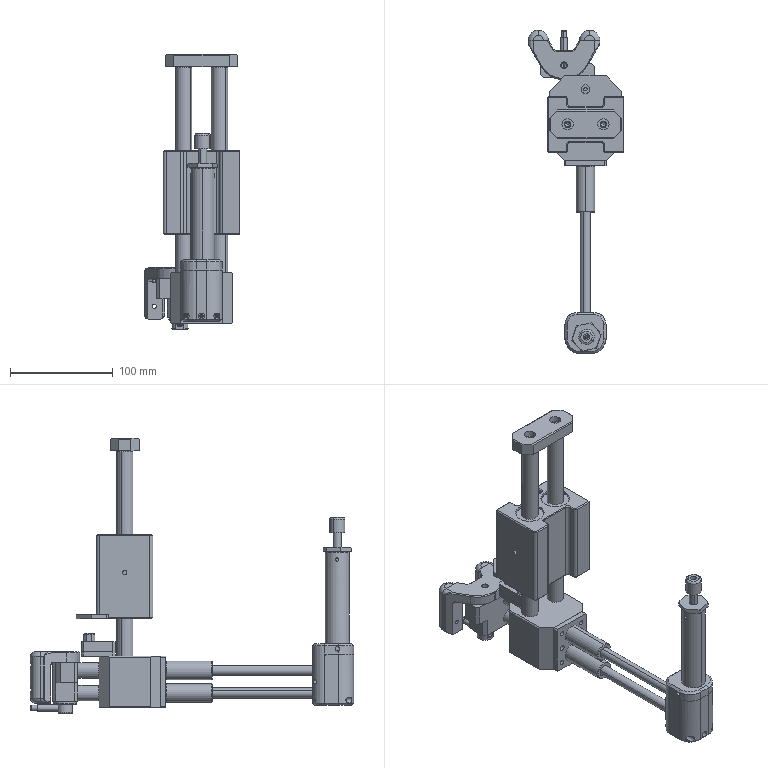Assembly | SolidWorks | mm | 37 component files | 38 solids | 1071 faces | box 93.5 x 315 x 268 mm | volume 759564 mm3 | cylinder 449 | plane 387 | cone 199 | torus 30 | spline 6 | commonest cylinder face diameters 4.2 x38 6 x38 10 x28 16 x27 4.5 x24 3.3 x22 5.5 x20 4 x20
Bill of materials:
DZ.KX.203-TC1505-20-18-05-90 | 1 | Plain Carbon Steel | Short thick-walled cylindrical sleeve with a stepped (counterbored) axial through bore and chamfered outer edges at both ends.
DZ.KX.203-TC1505-20-18-05-92 | 1 | Plain Carbon Steel | Solid cylinder with a small central axial through hole and a large rounded fillet on one end edge; other end appears square-edged.
DZ.KX.203-TC1505-20-18-05-93 | 1 | Plain Carbon Steel | Hex-flanged bushing: a hexagonal head with chamfered corners above a cylindrical shank, with a reduced-diameter neck/undercut directly under the head, a chamfered shank end, and a central axial through bore.
DZ.KX.203-TC1505-20-18-05-96 | 1 | Plain Carbon Steel | Slender stepped pin: a thin lower rod, a larger cylindrical collar, and an upper section of intermediate diameter with a small axial hole in its top end.
DZ.KX.203-TC1505-20-18-05-97 | 1 | Plain Carbon Steel | U-shaped channel/clip with a rounded back and two parallel side walls; inner wall profile has steps/notches, a slot cut into one leg near the bottom, several small holes near the bottom, and a chamfered bottom edge.
DZ.KX.203-TC1505-20-18-05-98 | 1 | Cast Stainless Steel | Long thin-walled tube with a small radial cross hole near one end and a short reduced-diameter groove/step near the other end; ends chamfered.
DZ.KX.203-TC1505-20-18-05-99 | 1 | Plain Carbon Steel | L-shaped bracket: a horizontal top ring with rounded-square outline and large circular bore, joined to a vertical plate with multiple holes.
DZ.KX.203-TC1505-30-09-01-05-01 | 1 |  | Rectangular block with an H-shaped plan profile (filleted rectangular recesses on two opposite sides), two parallel vertical through bores, and small holes on the side faces.
DZ.KX.203-TC1505-30-09-01-05-02 | 2 | Malleable Cast Iron | Long slender plain cylindrical rod with a small axial hole in one end and small end chamfers.
DZ.KX.203-TC1505-30-09-01-05-03 | 1 |  | Thin flat plate with an irregular polygonal outline (large chamfers on two upper corners, small on lower corners) and three through holes: one larger hole near the top center and two smaller holes near the lower corners.
DZ.KX.203-TC1505-30-09-01-05-05 | 1 | Plain Carbon Steel | Rectangular bar/plate with chamfered corners in plan (elongated octagon) and two counterbored through holes spaced along its length; top edges chamfered.
DZ.KX.203-TC1505-30-09-01-05-06 | 1 | 6061 Alloy | Near-cubic block with chamfered vertical edges, two counterbored holes and two small holes on the top face, two large through bores stacked on one side face surrounded by six small blind holes, and further holes on another face.
DZ.KX.203-TC1505-30-09-01-05-07 | 2 | Malleable Cast Iron | Long, slender straight cylindrical rod or tube with a small axial hole at the end.
DZ.KX.203-TC1505-30-09-01-05-08 | 1 |  | Flat rectangular plate with small corner chamfers, two large round through holes on the centerline and six smaller round through holes in two side columns of three.
DZ.KX.203-TC1505-30-09-01-05-10 | 1 | Plain Carbon Steel | Prismatic block with a stepped, chamfered outline, a large vertical through bore with an edge chamfer, and two counterbored horizontal holes through one side.
DZ.KX.203-TC1505-30-09-01-05-12 | 1 | Plain Carbon Steel | Stepped cylindrical pin: a longer large-diameter section and a shorter reduced-diameter end section, with chamfered ends and a small axial hole at the large end.
DZ.KX.203-TC1505-30-09-01-05-18 | 1 |  | Flanged bushing or spacer-like part: an upper body with two parallel flats, a wider base flange that also has two flats, chamfered edges and a small central through hole.
DZ.KX.203-TC1505-30-09-01-05-19 | 1 |  | Thick rectangular block with chamfered corners, one large through hole, four smaller through holes near the corners, and a rectangular channel cut across the underside.
DZ.KX.203-TC1505-30-09-01-05-20 | 1 |  | Thin flat rectangular plate with chamfered corners and four equal round through holes near the corners.
DZ.KX.203-TC1505-30-09-01-05-22 | 1 | Cast Carbon Steel | Cylindrical pin with an integral collar near one end, a small axial hole and flat or notch at the long end, and a cross hole through the short end, which also appears to have flats.
DZ.KX.203-TC1505-30-09-01-05-28 | 1 | Cast Carbon Steel | Bent bracket with a constant-thickness profile: a top plate with a rounded outer edge and a V-shaped notch with a flat bottom, plus two downward legs, each with two holes.
DZ.KX.203-TC1505-30-09-01-05-30 | 2 |  | Short thick-walled cylindrical tube or bushing with a large concentric through bore and small chamfers at the ends.
DZ.KX.203-TC1505-30-09-01-05-32 | 2 |  | Block with a half-round (D-shaped) profile, a flat face, two round holes through the flat face and rounded edges.
DZ.KX.203-TC1505-30-09-02-01-35 | 2 |  | Cylindrical tube or spacer with a concentric through bore and small chamfers at the ends; it is longer and more slender than unnamed part.
LMUW_N16 | 2 |  | Hollow straight cylindrical sleeve with a concentric through-bore and two shallow, narrow circumferential grooves, one near each end. Ends are flat annular faces with slight edge rounding or chamfers.
LMUW10 | 2 |  | Hollow straight cylindrical sleeve with a concentric through-bore and two shallow, narrow circumferential grooves near the ends. It is similar to the other part but looks slightly more slender.
SS_10GL2_ACTUATOR | 1 |  | Thin flat strip-like lever arm. One end has a short downturned lip. The other end has a U-shaped bracket with two upright side cheeks that hold a cylindrical roller on an axle pin; the pin sticks out past both cheeks.
SS_10GL2_BASE | 1 |  | Rectangular box-shaped body. A small rounded plunger nub sticks up from the top surface, which has a small raised step. Two round through-holes pass through the body sideways. Three thin flat blade-like pins stick out from the bottom edge.
TAC01-M4-L12 | 1 |  | Stepped cylindrical pin. It has a long, smaller-diameter shank and a larger-diameter head. A thin collar/flange, slightly wider than the head, sits where the shank meets the head. Both ends are chamfered.
YWY-D10-L35 | 1 |  | Helical coil spring made of round wire, with open coils of constant diameter. A short cylindrical ring/sleeve sits concentrically at one end. The free coil end at the other end is not closed.
Mates:
1. coincident | DZ.KX.203-TC1505-30-09-01-05-02-1 face at (277, -610.807, 213.06) dir (0, 0, 1) | DZ.KX.203-TC1505-30-09-01-05-02-2 face at (312, -610.807, 213.06) dir (0, 0, 1)
2. coincident | DZ.KX.203-TC1505-30-09-01-05-02-1 face at (277, -610.807, 213.06) dir (0, 0, 1) | DZ.KX.203-TC1505-30-09-01-05-05-1 face at (294.5, -610.807, 213.06) dir (0, 0, -1)
3. concentric | DZ.KX.203-TC1505-30-09-01-05-02-1 face at (277, -610.807, 213.06) dir (0, 0, -1) r 8 | DZ.KX.203-TC1505-30-09-01-05-05-1 face at (277, -610.807, 225.06) dir (0, 0, 1) r 5.5
4. concentric | DZ.KX.203-TC1505-30-09-01-05-02-2 face at (312, -610.807, 213.06) dir (0, 0, -1) r 8 | DZ.KX.203-TC1505-30-09-01-05-05-1 face at (312, -610.807, 225.06) dir (0, 0, 1) r 5.5
5. concentric | DZ.KX.203-TC1505-30-09-01-05-02-2 face at (312, -610.807, 213.06) dir (0, 0, -1) r 8 | DZ.KX.203-TC1505-30-09-01-05-06-1 face at (312, -610.807, -36.94) dir (0, 0, -1) r 5.5
6. concentric | DZ.KX.203-TC1505-30-09-01-05-02-1 face at (277, -610.807, 213.06) dir (0, 0, -1) r 8 | DZ.KX.203-TC1505-30-09-01-05-06-1 face at (277, -610.807, -36.94) dir (0, 0, -1) r 5.5
7. coincident | DZ.KX.203-TC1505-30-09-01-05-02-2 face at (312, -610.807, 8.06) dir (0, 0, -1) | DZ.KX.203-TC1505-30-09-01-05-06-1 face at (312, -610.807, 8.06) dir (0, 0, 1)
8. coincident | DZ.KX.203-TC1505-30-09-01-05-07-1 face at (294.5, -796.807, -0.9405) dir (0, -1, 0) | DZ.KX.203-TC1505-30-09-01-05-07-2 face at (294.5, -796.807, -22.94) dir (0, -1, 0)
9. coincident | DZ.KX.203-TC1505-30-09-01-05-06-1 face at (324.5, -645.807, 13.06) dir (0, -1, 0) | DZ.KX.203-TC1505-30-09-01-05-08-1 face at (294.5, -645.807, -11.94) dir (0, 1, 0)
10. distance | DZ.KX.203-TC1505-30-09-01-05-06-1 face at (324.5, -645.807, 13.06) dir (1, 0, 0) | DZ.KX.203-TC1505-30-09-01-05-08-1 face at (314.5, -645.807, -36.94) dir (1, 0, 0)
11. coincident | DZ.KX.203-TC1505-30-09-01-05-06-1 face at (294.5, -615.807, 13.06) dir (0, 0, 1) | DZ.KX.203-TC1505-30-09-01-05-08-1 face at (314.5, -645.807, 13.06) dir (0, 0, 1)
12. distance | DZ.KX.203-TC1505-30-09-01-05-06-1 face at (294.5, -615.807, 13.06) dir (0, 0, 1) | DZ.KX.203-TC1505-30-09-01-05-19-1 face at (313.5, -568.307, 17.06) dir (0, 0, -1)
13. concentric | DZ.KX.203-TC1505-30-09-01-05-18-1 face at (294.5, -576.307, 27.06) dir (0, 0, -1) r 6 | DZ.KX.203-TC1505-30-09-01-05-19-1 face at (294.5, -576.307, 17.06) dir (0, 0, 1) r 6.5
14. parallel | DZ.KX.203-TC1505-30-09-01-05-06-1 face at (324.5, -585.807, 13.06) dir (0, 1, 0) | DZ.KX.203-TC1505-30-09-01-05-19-1 face at (277.5, -568.307, 17.06) dir (0, 1, 0)
15. parallel | DZ.KX.203-TC1505-30-09-01-05-18-1 face at (288, -592.307, 21.06) dir (-1, 0, 0) | DZ.KX.203-TC1505-30-09-01-05-19-1 face at (287.5, -584.307, 21.06) dir (1, 0, 0)
16. coincident | DZ.KX.203-TC1505-30-09-01-05-18-1 face at (294.5, -576.307, 17.06) dir (0, 0, -1) | DZ.KX.203-TC1505-30-09-01-05-19-1 face at (313.5, -568.307, 17.06) dir (0, 0, -1)
17. coincident | DZ.KX.203-TC1505-30-09-01-05-19-1 face at (313.5, -568.307, 17.06) dir (0, 0, -1) | DZ.KX.203-TC1505-30-09-01-05-20-1 face at (294.5, -584.807, 17.06) dir (0, 0, 1)
18. coincident | DZ.KX.203-TC1505-30-09-01-05-19-1 face at (277.5, -568.307, 17.06) dir (0, 1, 0) | DZ.KX.203-TC1505-30-09-01-05-20-1 face at (313.5, -568.307, 17.06) dir (0, 1, 0)
19. coincident | DZ.KX.203-TC1505-30-09-01-05-19-1 face at (275.5, -582.307, 17.06) dir (-1, 0, 0) | DZ.KX.203-TC1505-30-09-01-05-20-1 face at (275.5, -601.307, 17.06) dir (-1, 0, 0)
20. concentric | DZ.KX.203-TC1505-30-09-01-05-07-1 face at (294.5, -561.807, -0.9405) dir (0, -1, 0) r 5 | DZ.KX.203-TC1505-30-09-01-05-06-1 face at (294.5, -645.807, -0.9405) dir (0, -1, 0) r 6
21. concentric | DZ.KX.203-TC1505-30-09-01-05-06-1 face at (294.5, -645.807, -22.94) dir (0, -1, 0) r 6 | DZ.KX.203-TC1505-30-09-01-05-07-2 face at (294.5, -561.807, -22.94) dir (0, -1, 0) r 5
22. coincident | DZ.KX.203-TC1505-30-09-01-05-06-1 edge at (294.5, -590.807, -0.9405) dir (0, -1, 0) r 9.5 | LMUW10-1 face at (289.5, -590.807, -0.9405) dir (0, 1, 0)
23. coincident | DZ.KX.203-TC1505-30-09-01-05-06-1 edge at (294.5, -590.807, -0.9405) dir (0, -1, 0) r 9.5 | LMUW10-1 face at (294.5, -618.307, -0.9405) dir (0, -1, 0) r 9.5
24. concentric | DZ.KX.203-TC1505-30-09-01-05-07-2 face at (294.5, -561.807, -22.94) dir (0, -1, 0) r 5 | LMUW10-3 face at (294.5, -618.307, -22.94) dir (0, -1, 0) r 9.5
25. coincident | DZ.KX.203-TC1505-30-09-01-05-06-1 edge at (294.5, -590.807, -22.94) dir (0, -1, 0) r 9.5 | LMUW10-3 face at (289.5, -590.807, -22.94) dir (0, 1, 0)
26. distance | DZ.KX.203-TC1505-30-09-01-05-20-1 face at (275.5, -601.307, 17.06) dir (-1, 0, 0) | DZ.KX.203-TC1505-30-09-01-05-06-1 face at (264.5, -645.807, 13.06) dir (-1, 0, 0)
27. distance | DZ.KX.203-TC1505-30-09-01-05-20-1 face at (313.5, -601.307, 17.06) dir (0, -1, 0) | DZ.KX.203-TC1505-30-09-01-05-06-1 face at (324.5, -585.807, 13.06) dir (0, 1, 0)
28. coincident | DZ.KX.203-TC1505-30-09-01-05-08-1 face at (294.5, -650.807, -11.94) dir (0, -1, 0) | DZ.KX.203-TC1505-30-09-02-01-35-1 face at (294.5, -650.807, -0.9405) dir (0, 1, 0)
29. concentric | DZ.KX.203-TC1505-30-09-01-05-07-1 face at (294.5, -561.807, -0.9405) dir (0, -1, 0) r 5 | DZ.KX.203-TC1505-30-09-02-01-35-1 face at (294.5, -650.807, -0.9405) dir (0, -1, 0) r 9
30. coincident | DZ.KX.203-TC1505-30-09-01-05-08-1 face at (294.5, -650.807, -11.94) dir (0, -1, 0) | DZ.KX.203-TC1505-30-09-02-01-35-2 face at (294.5, -650.807, -22.94) dir (0, 1, 0)
31. concentric | DZ.KX.203-TC1505-30-09-01-05-07-2 face at (294.5, -561.807, -22.94) dir (0, -1, 0) r 5 | DZ.KX.203-TC1505-30-09-02-01-35-2 face at (294.5, -650.807, -22.94) dir (0, -1, 0) r 9
32. coincident | DZ.KX.203-TC1505-30-09-01-05-03-4 face at (294.5, -579.307, 53.441) dir (0, 0, 1) | DZ.KX.203-TC1505-30-09-01-05-01-2 face at (257, -610.807, 53.441) dir (0, 0, -1)
33. concentric | DZ.KX.203-TC1505-30-09-01-05-03-4 face at (319.5, -589.307, 49.441) dir (0, 0, -1) r 2.75 | DZ.KX.203-TC1505-30-09-01-05-01-2 face at (319.5, -589.307, 53.441) dir (0, 0, -1) r 2.1
34. concentric | DZ.KX.203-TC1505-30-09-01-05-03-4 face at (269.5, -589.307, 49.441) dir (0, 0, -1) r 2.75 | DZ.KX.203-TC1505-30-09-01-05-01-2 face at (269.5, -589.307, 53.441) dir (0, 0, -1) r 2.1
35. coincident | LMUW_N16-3 face at (319.701, -608.64, 59.441) dir (0, 0, -1) | DZ.KX.203-TC1505-30-09-01-05-01-2 face at (322, -610.807, 59.441) dir (0, 0, 1)
36. concentric | LMUW_N16-3 face at (312, -610.807, 94.441) dir (0, 0, 1) r 14 | DZ.KX.203-TC1505-30-09-01-05-01-2 face at (312, -610.807, 131.441) dir (0, 0, 1) r 14
37. coincident | LMUW_N16-3 face at (324.707, -607.232, 129.441) dir (0, 0, 1) | LMUW_N16-4 face at (289.707, -607.232, 129.441) dir (0, 0, 1)
38. concentric | DZ.KX.203-TC1505-30-09-01-05-01-2 face at (277, -610.807, 131.441) dir (0, 0, 1) r 14 | LMUW_N16-4 face at (277, -610.807, 94.441) dir (0, 0, 1) r 14
39. concentric | DZ.KX.203-TC1505-30-09-01-05-02-1 face at (277, -610.807, 213.06) dir (0, 0, -1) r 8 | DZ.KX.203-TC1505-30-09-01-05-01-2 face at (277, -610.807, 131.441) dir (0, 0, 1) r 14
40. concentric | DZ.KX.203-TC1505-30-09-01-05-02-2 face at (312, -610.807, 213.06) dir (0, 0, -1) r 8 | DZ.KX.203-TC1505-30-09-01-05-01-2 face at (312, -610.807, 131.441) dir (0, 0, 1) r 14
41. coincident | DZ.KX.203-TC1505-30-09-01-05-07-1 face at (294.5, -561.807, -0.9405) dir (0, 1, 0) | DZ.KX.203-TC1505-30-09-01-05-10-1 face at (294.5, -561.807, -0.9405) dir (0, -1, 0)
42. concentric | DZ.KX.203-TC1505-30-09-01-05-07-1 face at (294.5, -561.807, -0.9405) dir (0, -1, 0) r 5 | DZ.KX.203-TC1505-30-09-01-05-10-1 face at (294.5, -550.807, -0.9405) dir (0, 1, 0) r 3.75
43. concentric | DZ.KX.203-TC1505-30-09-01-05-07-2 face at (294.5, -561.807, -22.94) dir (0, -1, 0) r 5 | DZ.KX.203-TC1505-30-09-01-05-10-1 face at (294.5, -550.807, -22.94) dir (0, 1, 0) r 3.75
44. concentric | DZ.KX.203-TC1505-30-09-01-05-10-1 face at (273.5, -552.807, 7.06) dir (0, 0, 1) r 8 | DZ.KX.203-TC1505-30-09-01-05-22-2 face at (273.5, -552.807, 4.16) dir (0, 0, -1) r 8
45. concentric | DZ.KX.203-TC1505-30-09-01-05-12-1 face at (273.5, -552.807, -37.44) dir (0, 1, 0) r 3.25 | DZ.KX.203-TC1505-30-09-01-05-22-2 face at (273.5, -545.807, -37.44) dir (0, 1, 0) r 3.25
46. coincident | DZ.KX.203-TC1505-30-09-01-05-28-2 face at (236.561, -528.807, 17.16) dir (0, 1, 0) | DZ.KX.203-TC1505-30-09-01-05-32-2 face at (288.5, -528.807, -32.84) dir (0, -1, 0)
47. coincident | DZ.KX.203-TC1505-30-09-01-05-28-2 face at (288.5, -566.807, -32.84) dir (0, 0, -1) | DZ.KX.203-TC1505-30-09-01-05-32-2 face at (298.5, -528.807, -32.84) dir (0, 0, -1)
48. coincident | DZ.KX.203-TC1505-30-09-01-05-28-2 face at (308.5, -592.04, -32.84) dir (1, 0, 0) | DZ.KX.203-TC1505-30-09-01-05-32-2 edge at (308.5, -528.807, -27.84) dir (0, 0, 1)
49. coincident | DZ.KX.203-TC1505-30-09-01-05-28-2 face at (236.561, -528.807, 17.16) dir (0, 1, 0) | DZ.KX.203-TC1505-30-09-01-05-32-3 face at (238.5, -528.807, -32.84) dir (0, -1, 0)
50. coincident | DZ.KX.203-TC1505-30-09-01-05-28-2 face at (288.5, -566.807, 17.16) dir (0, 0, 1) | DZ.KX.203-TC1505-30-09-01-05-32-3 face at (248.5, -528.807, 17.16) dir (0, 0, 1)
51. coincident | DZ.KX.203-TC1505-30-09-01-05-28-2 face at (238.5, -592.04, -32.84) dir (-1, 0, 0) | DZ.KX.203-TC1505-30-09-01-05-32-3 edge at (238.5, -528.807, -27.84) dir (0, 0, 1)
52. concentric | DZ.KX.203-TC1505-30-09-01-05-22-2 face at (273.5, -552.807, 4.16) dir (0, 0, -1) r 8 | DZ.KX.203-TC1505-30-09-01-05-28-2 face at (273.5, -552.807, 17.16) dir (0, 0, -1) r 8
53. coincident | DZ.KX.203-TC1505-30-09-01-05-06-1 face at (324.5, -585.807, 13.06) dir (0, 1, 0) | DZ.KX.203-TC1505-30-09-01-05-30-4 face at (294.5, -585.807, -0.9405) dir (0, -1, 0)
54. concentric | DZ.KX.203-TC1505-30-09-01-05-07-1 face at (294.5, -561.807, -0.9405) dir (0, -1, 0) r 5 | DZ.KX.203-TC1505-30-09-01-05-30-4 face at (294.5, -564.807, -0.9405) dir (0, -1, 0) r 7.75
55. coincident | TAC01-M4-L12-2 face at (248.5, -524.807, 4.66) dir (0, -1, 0) | DZ.KX.203-TC1505-30-09-01-05-32-3 face at (248.5, -524.807, 2.41) dir (0, 1, 0)
56. concentric | TAC01-M4-L12-2 face at (248.5, -535.807, 4.66) dir (0, 1, 0) r 2 | DZ.KX.203-TC1505-30-09-01-05-32-3 face at (248.5, -518.807, 4.66) dir (0, 1, 0) r 3.75
57. coincident | DZ.KX.203-TC1505-30-09-01-05-06-1 face at (324.5, -585.807, 13.06) dir (0, 1, 0) | DZ.KX.203-TC1505-30-09-01-05-30-5 face at (294.5, -585.807, -22.94) dir (0, -1, 0)
58. concentric | DZ.KX.203-TC1505-30-09-01-05-07-2 face at (294.5, -561.807, -22.94) dir (0, -1, 0) r 5 | DZ.KX.203-TC1505-30-09-01-05-30-5 face at (294.5, -564.807, -22.94) dir (0, -1, 0) r 7.75
59. coincident | DZ.KX.203-TC1505-30-09-01-05-10-1 face at (303, -564.807, -30.94) dir (0, -1, 0) | DZ.KX.203-TC1505-30-09-01-05-30-4 face at (294.5, -564.807, -0.9405) dir (0, 1, 0)
60. coincident | DZ.KX.203-TC1505-30-09-01-05-12-1 face at (273.5, -552.807, -37.44) dir (0, -1, 0) | DZ.KX.203-TC1505-30-09-01-05-22-2 face at (273.5, -552.807, -37.44) dir (0, 1, 0)
61. coincident | DZ.KX.203-TC1505-30-09-01-05-10-1 face at (303, -550.807, -30.94) dir (0, 0, -1) | DZ.KX.203-TC1505-30-09-01-05-22-2 face at (273.5, -552.807, -30.94) dir (0, 0, 1)
62. coincident | DZ.KX.203-TC1505-30-09-01-05-22-2 face at (266.5, -530.337, 7.16) dir (-1, 0, 0) | DZ.KX.203-TC1505-30-09-01-05-28-2 face at (266.5, -548.934, 17.16) dir (1, 0, 0)
63. coincident | DZ.KX.203-TC1505-30-09-01-05-22-2 face at (273.5, -552.807, 12.16) dir (0, 0, 1) | DZ.KX.203-TC1505-30-09-01-05-28-2 face at (273.5, -552.807, 12.16) dir (0, 0, -1)
64. angle | DZ.KX.203-TC1505-30-09-01-05-28-2 face at (310.439, -528.807, 17.16) dir (0.866, -0.5, 0) | DZ.KX.203-TC1505-30-09-01-05-10-1 face at (303, -550.807, -30.94) dir (1, 0, 0)
65. coincident | DZ.KX.203-TC1505-30-09-01-05-07-2 face at (294.5, -796.807, -22.94) dir (0, -1, 0) | DZ.KX.203-TC1505-20-18-05-99-1 face at (294.5, -796.807, -22.94) dir (0, 1, 0)
66. concentric | DZ.KX.203-TC1505-30-09-01-05-07-2 face at (294.5, -561.807, -22.94) dir (0, -1, 0) r 5 | DZ.KX.203-TC1505-20-18-05-99-1 face at (294.5, -805.807, -22.94) dir (0, -1, 0) r 3.75
67. concentric | DZ.KX.203-TC1505-30-09-01-05-07-1 face at (294.5, -561.807, -0.9405) dir (0, -1, 0) r 5 | DZ.KX.203-TC1505-20-18-05-99-1 face at (294.5, -805.807, -0.9405) dir (0, -1, 0) r 3.75
68. distance | SS_10GL2-1/SS_10GL2_BASE-1 face at (293.7, -821.107, -9.94) dir (0, 0, -1) | DZ.KX.203-TC1505-20-18-05-99-1 face at (274.5, -805.807, -34.94) dir (0, 0, -1)
69. distance | SS_10GL2-1/SS_10GL2_BASE-1 face at (297.5, -821.107, -0.04045) dir (1, 0, 0) | DZ.KX.203-TC1505-20-18-05-99-1 face at (314.5, -805.807, -34.94) dir (1, 0, 0)
70. coincident | DZ.KX.203-TC1505-20-18-05-99-1 face at (294.5, -805.807, -9.94) dir (0, -1, 0) | DZ.KX.203-TC1505-20-18-05-97-1 face at (294.5, -805.807, -9.94) dir (0, 1, 0)
71. coincident | DZ.KX.203-TC1505-20-18-05-99-1 face at (274.5, -805.807, -34.94) dir (-1, 0, 0) | DZ.KX.203-TC1505-20-18-05-97-1 face at (274.5, -833.807, -34.94) dir (-1, 0, 0)
72. coincident | SS_10GL2-1/SS_10GL2_BASE-1 face at (297.5, -821.107, -9.54) dir (0, -1, 0) | DZ.KX.203-TC1505-20-18-05-97-1 face at (280, -821.107, -22.94) dir (0, 1, 0)
73. concentric | DZ.KX.203-TC1505-20-18-05-98-1 face at (295.5, -817.807, 115.06) dir (0, 0, 1) r 6.1 | DZ.KX.203-TC1505-20-18-05-96-1 face at (295.5, -817.807, 24.06) dir (0, 0, -1) r 6
74. coincident | DZ.KX.203-TC1505-20-18-05-98-1 edge at (295.5, -817.807, 55.06) dir (0, 0, 1) r 6.1 | YWY-D10-L35-1 face at (295.5, -817.807, 55.06) dir (0, 0, -1)
75. concentric | DZ.KX.203-TC1505-20-18-05-96-1 face at (295.5, -817.807, 24.06) dir (0, 0, -1) r 3 | YWY-D10-L35-1 face at (295.5, -817.807, 58.06) dir (0, 0, -1) r 5
76. coincident | DZ.KX.203-TC1505-20-18-05-99-1 face at (274.5, -805.807, -34.94) dir (0, 0, -1) | DZ.KX.203-TC1505-20-18-05-97-1 face at (274.5, -833.807, -34.94) dir (0, 0, -1)
77. concentric | DZ.KX.203-TC1505-20-18-05-99-1 face at (295.5, -817.807, 25.06) dir (0, 0, 1) r 11.5 | DZ.KX.203-TC1505-20-18-05-98-1 face at (295.5, -817.807, 15.06) dir (0, 0, 1) r 11.5
78. coincident | DZ.KX.203-TC1505-20-18-05-99-1 face at (294.5, -793.807, 15.06) dir (0, 0, -1) | DZ.KX.203-TC1505-20-18-05-98-1 face at (295.5, -817.807, 15.06) dir (0, 0, -1)
79. coincident | DZ.KX.203-TC1505-20-18-05-98-1 face at (295.5, -817.807, 115.06) dir (0, 0, 1) | DZ.KX.203-TC1505-20-18-05-93-1 face at (295.5, -817.807, 115.06) dir (0, 0, -1)
80. concentric | DZ.KX.203-TC1505-20-18-05-98-1 face at (295.5, -817.807, 15.06) dir (0, 0, 1) r 11.5 | DZ.KX.203-TC1505-20-18-05-93-1 face at (295.5, -817.807, 103.06) dir (0, 0, 1) r 8
81. concentric | DZ.KX.203-TC1505-20-18-05-96-1 face at (295.5, -817.807, 24.06) dir (0, 0, -1) r 4 | DZ.KX.203-TC1505-20-18-05-92-1 face at (295.5, -817.807, 133.06) dir (0, 0, -1) r 4
82. coincident | DZ.KX.203-TC1505-20-18-05-96-1 face at (295.5, -817.807, 138.06) dir (0, 0, 1) | DZ.KX.203-TC1505-20-18-05-92-1 face at (295.5, -817.807, 138.06) dir (0, 0, -1)
83. coincident | DZ.KX.203-TC1505-20-18-05-96-1 face at (296.925, -815.167, 24.06) dir (0, 0, -1) | DZ.KX.203-TC1505-20-18-05-90-1 face at (295.5, -817.807, 24.06) dir (0, 0, 1)
84. concentric | DZ.KX.203-TC1505-20-18-05-96-1 face at (295.5, -817.807, 24.06) dir (0, 0, -1) r 3 | DZ.KX.203-TC1505-20-18-05-90-1 face at (295.5, -817.807, 27.06) dir (0, 0, -1) r 5